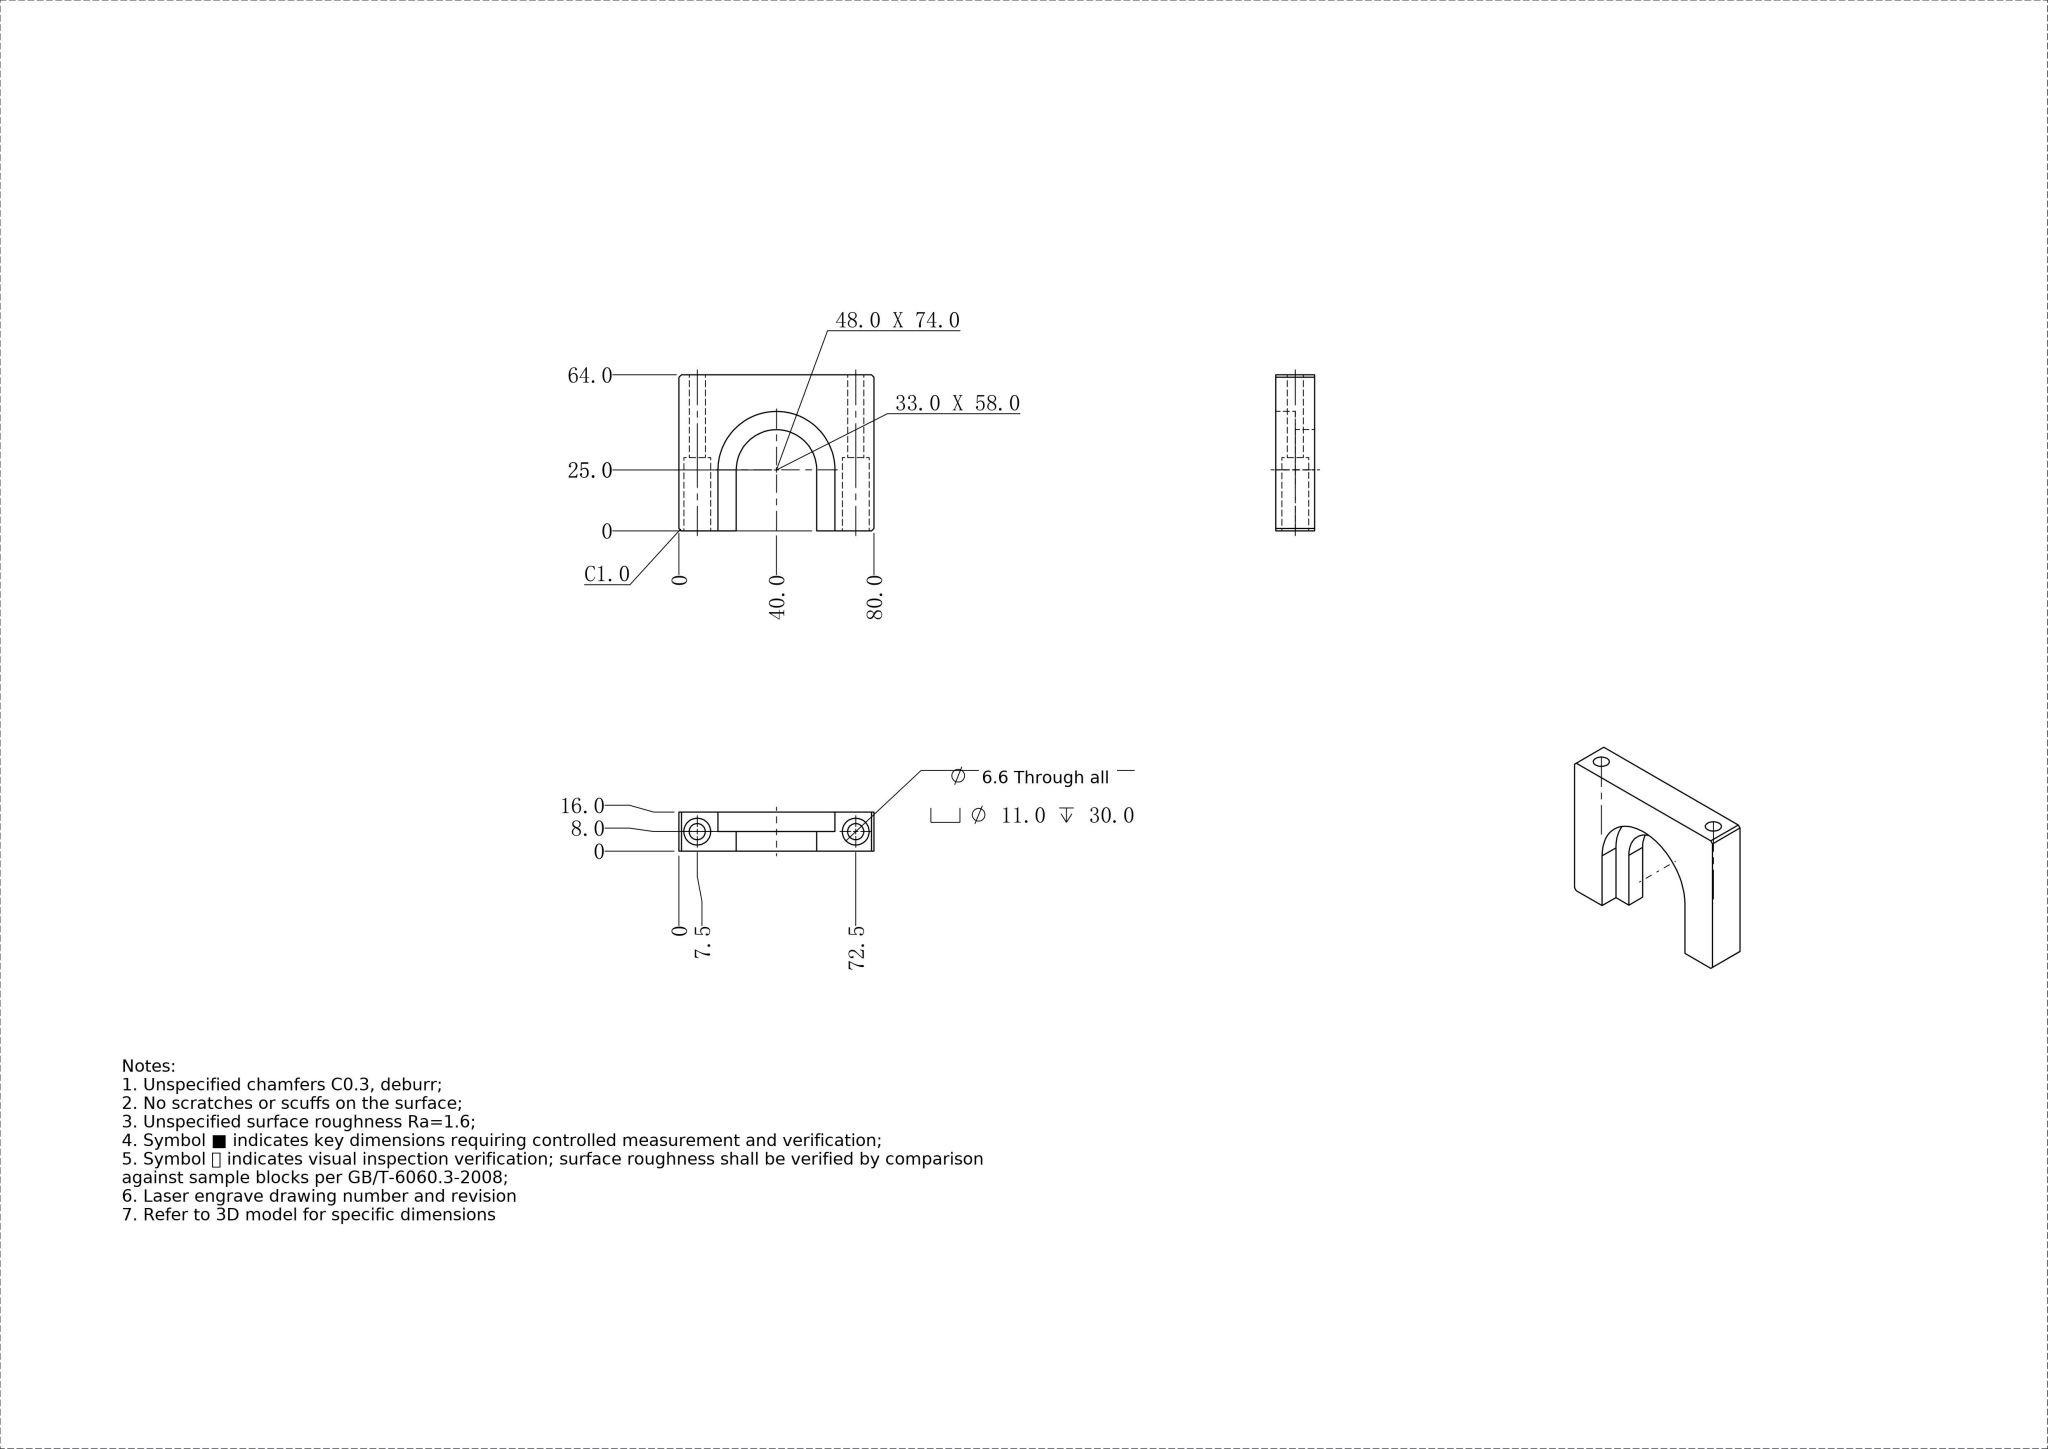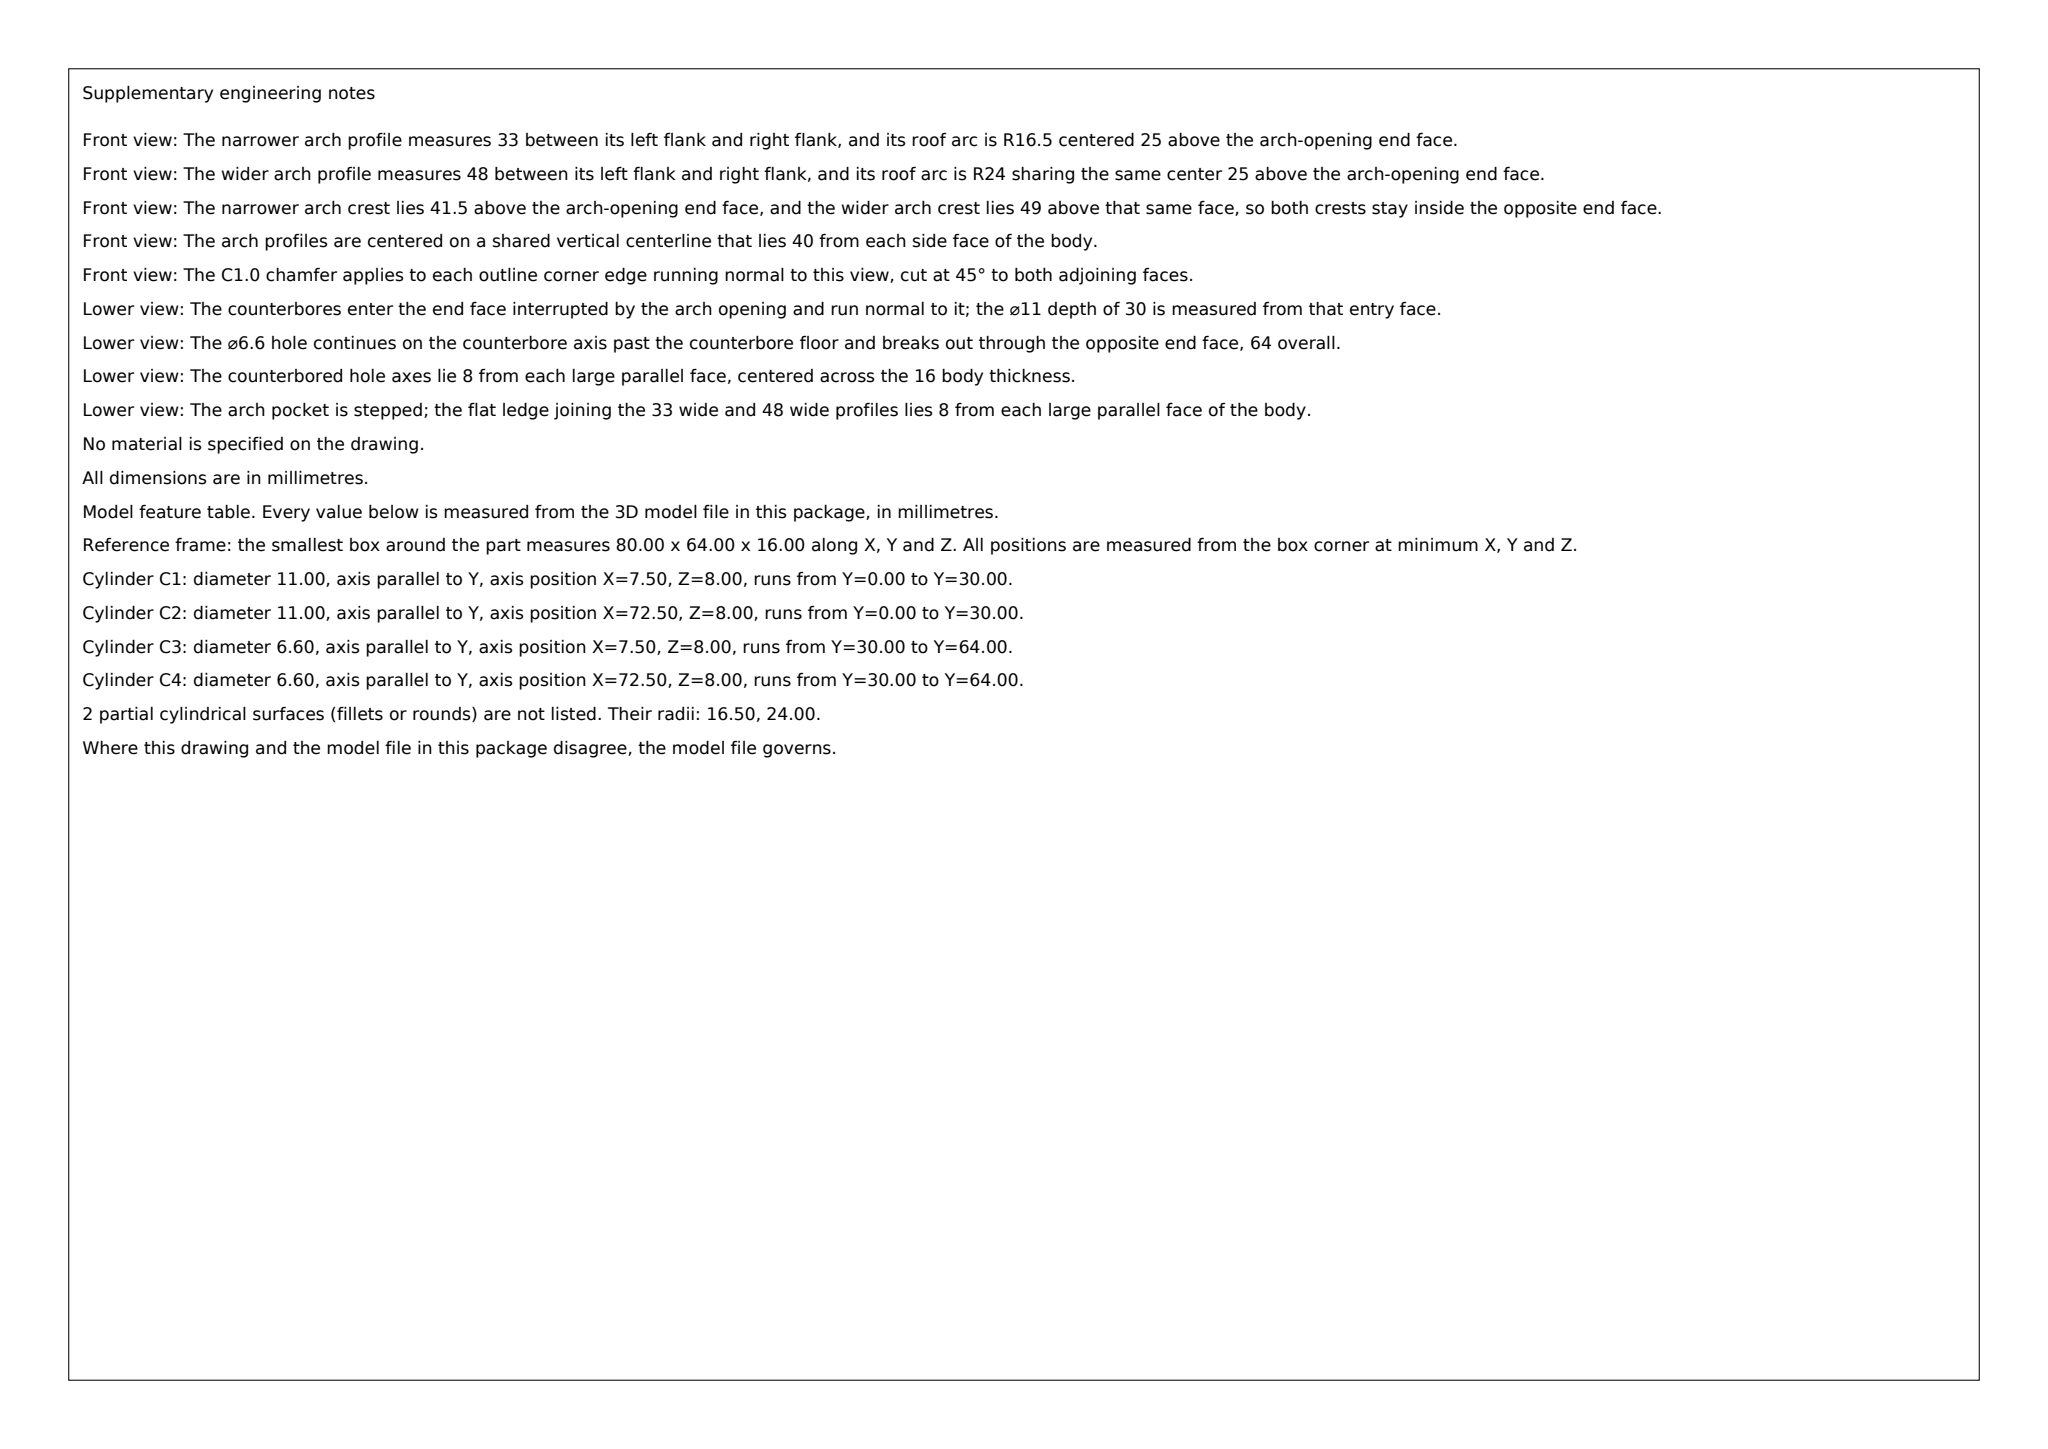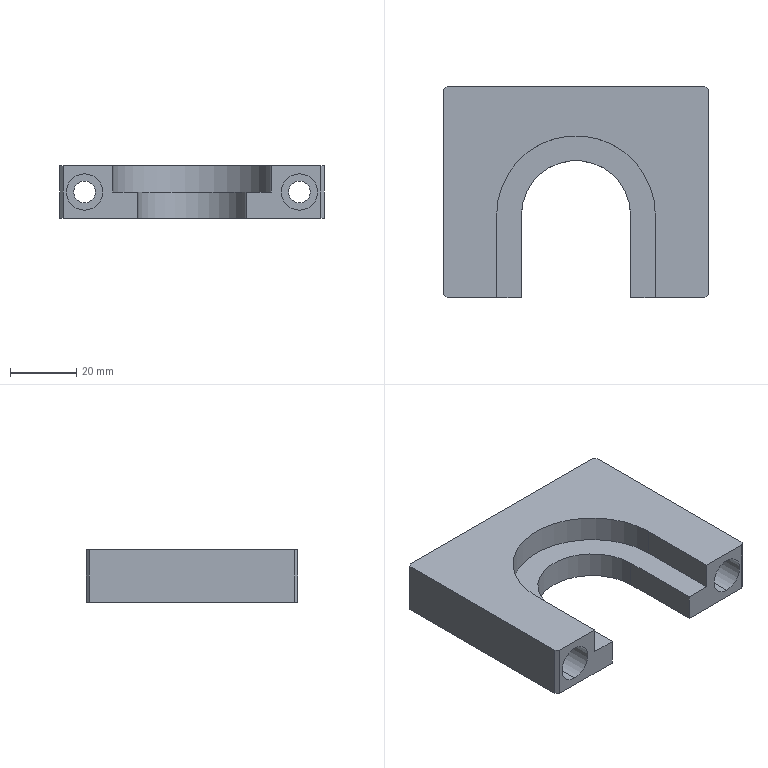Part | SolidWorks | mm | 1 solid | 28 faces | box 80 x 64 x 16 mm | volume 47000 mm3 | plane 18 | cylinder 10 | commonest cylinder face diameters 11 x4 6.6 x4 33 x1 48 x1
Drawing notes:
ALL DIMS IN MM UNLESS OTHERWISE NOTED | from the solid: STEP bbox 80.0 x 64.0 x 16.0 mm matches drawn 80.0/64.0/16.0 values
ARCH SLOTS Ø48.0 & Ø33.0 HT 8.0 EA, OPPOSITE FACES, THRU 16.0 | from the solid: cyl Ø48 axis z len 8 @ (40,25); cyl Ø33 axis z len 8 @ (40,25); z planes 0/8/16 in 16 thk plate
4X C1.0 CHAMFER ON ALL FOUR VERTICAL CORNER EDGES (AT X=0/80, Y=0/64), FULL 16.0 PART HEIGHT | from the solid: inclined_planes: four 45deg faces, size [1.0,1.0,16.0], bbox_from [0,0,0], [0,63,0], [79,0,0], [79,63,0]
build123d program:
from build123d import *

# Parameters (mm, degrees)
SKETCH1_W                                       = 80
SKETCH1_H                                       = 64
BOSS_EXTRUDE1_DEPTH                             = 16
CUT_EXTRUDE1_DEPTH                              = 16
CUT_EXTRUDE2_DEPTH                              = 8
M6_HEX_SOCKET_HEAD_CAP_SCREW_CBORE1_D           = 6.6
M6_HEX_SOCKET_HEAD_CAP_SCREW_CBORE1_CBORE_D     = 11
M6_HEX_SOCKET_HEAD_CAP_SCREW_CBORE1_CBORE_DEPTH = 30
CHAMFER1_SIZE                                   = 1


with BuildPart() as part:
    # Sketch1 → Boss-Extrude1 (new body)
    with BuildSketch(Plane.XY):
        Rectangle(SKETCH1_W, SKETCH1_H)
    extrude(amount=BOSS_EXTRUDE1_DEPTH)

    # Sketch2 → Cut-Extrude1 (cut)
    with BuildSketch(Plane.XY.offset(16)):
        with BuildLine():
            Line((-16.5, -32), (-16.5, -7))
            ThreePointArc((-16.5, -7), (0, 9.5), (16.5, -7))
            Line((16.5, -7), (16.5, -32))
            ThreePointArc((16.5, -32), (0, -48.5), (-16.5, -32))
        make_face()
    extrude(amount=-CUT_EXTRUDE1_DEPTH, mode=Mode.SUBTRACT)

    # Sketch3 → Cut-Extrude2 (cut)
    with BuildSketch(Plane.XY.offset(16)):
        with BuildLine():
            Line((24, -7), (24, -33))
            ThreePointArc((24, -33), (0, -57), (-24, -33))
            Line((-24, -33), (-24, -7))
            ThreePointArc((-24, -7), (0, 17), (24, -7))
        make_face()
    extrude(amount=-CUT_EXTRUDE2_DEPTH, mode=Mode.SUBTRACT)

    # M6 Hex Socket Head Cap Screw CBORE1 (through all)
    with Locations(Plane(origin=(0, -32, 0), x_dir=(-1, 0, 0), z_dir=(0, -1, 0))):
        with Locations((-32.5, -8), (32.5, -8)):
            CounterBoreHole(M6_HEX_SOCKET_HEAD_CAP_SCREW_CBORE1_D / 2, M6_HEX_SOCKET_HEAD_CAP_SCREW_CBORE1_CBORE_D / 2, M6_HEX_SOCKET_HEAD_CAP_SCREW_CBORE1_CBORE_DEPTH)

    # Chamfer1
    chamfer1_edges = [part.edges().sort_by_distance(p)[0] for p in [
        (40, -32, 8),
        (-40, -32, 8),
        (-40, 32, 8),
        (40, 32, 8),
    ]]
    chamfer(chamfer1_edges, length=CHAMFER1_SIZE)


solid = part.part
STEP:
#1=CARTESIAN_POINT('',(32.5,-2.,13.5));
#2=VERTEX_POINT('',#1);
#3=CARTESIAN_POINT('',(32.5,-2.,2.5));
#4=VERTEX_POINT('',#3);
#5=CARTESIAN_POINT('',(32.5,-2.,8.));
#6=DIRECTION('',(0.,-1.,0.));
#7=DIRECTION('',(0.,0.,-1.));
#8=AXIS2_PLACEMENT_3D('',#5,#6,#7);
#9=CIRCLE('',#8,5.5);
#10=EDGE_CURVE('',#2,#4,#9,.T.);
#11=ORIENTED_EDGE('',*,*,#10,.F.);
#12=CARTESIAN_POINT('',(32.5,-32.,13.5));
#13=VERTEX_POINT('',#12);
#14=CARTESIAN_POINT('',(32.5,-32.,13.5));
#15=DIRECTION('',(0.,-1.,0.));
#16=VECTOR('',#15,1000.);
#17=LINE('',#14,#16);
#18=EDGE_CURVE('',#2,#13,#17,.T.);
#19=ORIENTED_EDGE('',*,*,#18,.T.);
#20=CARTESIAN_POINT('',(32.5,-32.,2.5));
#21=VERTEX_POINT('',#20);
#22=CARTESIAN_POINT('',(32.5,-32.,8.));
#23=DIRECTION('',(0.,-1.,0.));
#24=DIRECTION('',(0.,0.,-1.));
#25=AXIS2_PLACEMENT_3D('',#22,#23,#24);
#26=CIRCLE('',#25,5.5);
#27=EDGE_CURVE('',#13,#21,#26,.T.);
#28=ORIENTED_EDGE('',*,*,#27,.T.);
#29=CARTESIAN_POINT('',(32.5,-32.,2.5));
#30=DIRECTION('',(0.,-1.,0.));
#31=VECTOR('',#30,1000.);
#32=LINE('',#29,#31);
#33=EDGE_CURVE('',#4,#21,#32,.T.);
#34=ORIENTED_EDGE('',*,*,#33,.F.);
#35=EDGE_LOOP('',(#11,#19,#28,#34));
#36=FACE_OUTER_BOUND('',#35,.T.);
#37=CARTESIAN_POINT('',(32.5,-32.,8.));
#38=DIRECTION('',(0.,-1.,0.));
#39=DIRECTION('',(0.,0.,-1.));
#40=AXIS2_PLACEMENT_3D('',#37,#38,#39);
#41=CYLINDRICAL_SURFACE('',#40,5.5);
#42=ADVANCED_FACE('',(#36),#41,.F.);
#43=CARTESIAN_POINT('',(32.5,32.,11.3));
#44=VERTEX_POINT('',#43);
#45=CARTESIAN_POINT('',(32.5,32.,4.7));
#46=VERTEX_POINT('',#45);
#47=CARTESIAN_POINT('',(32.5,32.,8.));
#48=DIRECTION('',(0.,-1.,0.));
#49=DIRECTION('',(0.,0.,-1.));
#50=AXIS2_PLACEMENT_3D('',#47,#48,#49);
#51=CIRCLE('',#50,3.3);
#52=EDGE_CURVE('',#44,#46,#51,.T.);
#53=ORIENTED_EDGE('',*,*,#52,.F.);
#54=CARTESIAN_POINT('',(32.5,-2.,11.3));
#55=VERTEX_POINT('',#54);
#56=CARTESIAN_POINT('',(32.5,-32.,11.3));
#57=DIRECTION('',(0.,-1.,0.));
#58=VECTOR('',#57,1000.);
#59=LINE('',#56,#58);
#60=EDGE_CURVE('',#44,#55,#59,.T.);
#61=ORIENTED_EDGE('',*,*,#60,.T.);
#62=CARTESIAN_POINT('',(32.5,-2.,4.7));
#63=VERTEX_POINT('',#62);
#64=CARTESIAN_POINT('',(32.5,-2.,8.));
#65=DIRECTION('',(0.,-1.,0.));
#66=DIRECTION('',(0.,0.,-1.));
#67=AXIS2_PLACEMENT_3D('',#64,#65,#66);
#68=CIRCLE('',#67,3.3);
#69=EDGE_CURVE('',#55,#63,#68,.T.);
#70=ORIENTED_EDGE('',*,*,#69,.T.);
#71=CARTESIAN_POINT('',(32.5,-32.,4.7));
#72=DIRECTION('',(0.,-1.,0.));
#73=VECTOR('',#72,1000.);
#74=LINE('',#71,#73);
#75=EDGE_CURVE('',#46,#63,#74,.T.);
#76=ORIENTED_EDGE('',*,*,#75,.F.);
#77=EDGE_LOOP('',(#53,#61,#70,#76));
#78=FACE_OUTER_BOUND('',#77,.T.);
#79=CARTESIAN_POINT('',(32.5,-32.,8.));
#80=DIRECTION('',(0.,-1.,0.));
#81=DIRECTION('',(0.,0.,-1.));
#82=AXIS2_PLACEMENT_3D('',#79,#80,#81);
#83=CYLINDRICAL_SURFACE('',#82,3.3);
#84=ADVANCED_FACE('',(#78),#83,.F.);
#85=CARTESIAN_POINT('',(-32.5,-2.,13.5));
#86=VERTEX_POINT('',#85);
#87=CARTESIAN_POINT('',(-32.5,-2.,2.5));
#88=VERTEX_POINT('',#87);
#89=CARTESIAN_POINT('',(-32.5,-2.,8.));
#90=DIRECTION('',(0.,-1.,0.));
#91=DIRECTION('',(0.,0.,-1.));
#92=AXIS2_PLACEMENT_3D('',#89,#90,#91);
#93=CIRCLE('',#92,5.5);
#94=EDGE_CURVE('',#86,#88,#93,.T.);
#95=ORIENTED_EDGE('',*,*,#94,.F.);
#96=CARTESIAN_POINT('',(-32.5,-32.,13.5));
#97=VERTEX_POINT('',#96);
#98=CARTESIAN_POINT('',(-32.5,-32.,13.5));
#99=DIRECTION('',(0.,-1.,0.));
#100=VECTOR('',#99,1000.);
#101=LINE('',#98,#100);
#102=EDGE_CURVE('',#86,#97,#101,.T.);
#103=ORIENTED_EDGE('',*,*,#102,.T.);
#104=CARTESIAN_POINT('',(-32.5,-32.,2.5));
#105=VERTEX_POINT('',#104);
#106=CARTESIAN_POINT('',(-32.5,-32.,8.));
#107=DIRECTION('',(0.,-1.,0.));
#108=DIRECTION('',(0.,0.,-1.));
#109=AXIS2_PLACEMENT_3D('',#106,#107,#108);
#110=CIRCLE('',#109,5.5);
#111=EDGE_CURVE('',#97,#105,#110,.T.);
#112=ORIENTED_EDGE('',*,*,#111,.T.);
#113=CARTESIAN_POINT('',(-32.5,-32.,2.5));
#114=DIRECTION('',(0.,-1.,0.));
#115=VECTOR('',#114,1000.);
#116=LINE('',#113,#115);
#117=EDGE_CURVE('',#88,#105,#116,.T.);
#118=ORIENTED_EDGE('',*,*,#117,.F.);
#119=EDGE_LOOP('',(#95,#103,#112,#118));
#120=FACE_OUTER_BOUND('',#119,.T.);
#121=CARTESIAN_POINT('',(-32.5,-32.,8.));
#122=DIRECTION('',(0.,-1.,0.));
#123=DIRECTION('',(0.,0.,-1.));
#124=AXIS2_PLACEMENT_3D('',#121,#122,#123);
#125=CYLINDRICAL_SURFACE('',#124,5.5);
#126=ADVANCED_FACE('',(#120),#125,.F.);
#127=CARTESIAN_POINT('',(-32.5,32.,11.3));
#128=VERTEX_POINT('',#127);
#129=CARTESIAN_POINT('',(-32.5,32.,4.7));
#130=VERTEX_POINT('',#129);
#131=CARTESIAN_POINT('',(-32.5,32.,8.));
#132=DIRECTION('',(0.,-1.,0.));
#133=DIRECTION('',(0.,0.,-1.));
#134=AXIS2_PLACEMENT_3D('',#131,#132,#133);
#135=CIRCLE('',#134,3.3);
#136=EDGE_CURVE('',#128,#130,#135,.T.);
#137=ORIENTED_EDGE('',*,*,#136,.F.);
#138=CARTESIAN_POINT('',(-32.5,-2.,11.3));
#139=VERTEX_POINT('',#138);
#140=CARTESIAN_POINT('',(-32.5,-32.,11.3));
#141=DIRECTION('',(0.,-1.,0.));
#142=VECTOR('',#141,1000.);
#143=LINE('',#140,#142);
#144=EDGE_CURVE('',#128,#139,#143,.T.);
#145=ORIENTED_EDGE('',*,*,#144,.T.);
#146=CARTESIAN_POINT('',(-32.5,-2.,4.7));
#147=VERTEX_POINT('',#146);
#148=CARTESIAN_POINT('',(-32.5,-2.,8.));
#149=DIRECTION('',(0.,-1.,0.));
#150=DIRECTION('',(0.,0.,-1.));
#151=AXIS2_PLACEMENT_3D('',#148,#149,#150);
#152=CIRCLE('',#151,3.3);
#153=EDGE_CURVE('',#139,#147,#152,.T.);
#154=ORIENTED_EDGE('',*,*,#153,.T.);
#155=CARTESIAN_POINT('',(-32.5,-32.,4.7));
#156=DIRECTION('',(0.,-1.,0.));
#157=VECTOR('',#156,1000.);
#158=LINE('',#155,#157);
#159=EDGE_CURVE('',#130,#147,#158,.T.);
#160=ORIENTED_EDGE('',*,*,#159,.F.);
#161=EDGE_LOOP('',(#137,#145,#154,#160));
#162=FACE_OUTER_BOUND('',#161,.T.);
#163=CARTESIAN_POINT('',(-32.5,-32.,8.));
#164=DIRECTION('',(0.,-1.,0.));
#165=DIRECTION('',(0.,0.,-1.));
#166=AXIS2_PLACEMENT_3D('',#163,#164,#165);
#167=CYLINDRICAL_SURFACE('',#166,3.3);
#168=ADVANCED_FACE('',(#162),#167,.F.);
#169=CARTESIAN_POINT('',(-16.5,-32.,8.));
#170=VERTEX_POINT('',#169);
#171=CARTESIAN_POINT('',(-16.5,-7.,8.));
#172=VERTEX_POINT('',#171);
#173=CARTESIAN_POINT('',(-16.5,-32.,8.));
#174=DIRECTION('',(0.,1.,0.));
#175=VECTOR('',#174,1000.);
#176=LINE('',#173,#175);
#177=EDGE_CURVE('',#170,#172,#176,.T.);
#178=ORIENTED_EDGE('',*,*,#177,.F.);
#179=CARTESIAN_POINT('',(-16.5,-32.,0.));
#180=VERTEX_POINT('',#179);
#181=CARTESIAN_POINT('',(-16.5,-32.,0.));
#182=DIRECTION('',(0.,0.,1.));
#183=VECTOR('',#182,1000.);
#184=LINE('',#181,#183);
#185=EDGE_CURVE('',#180,#170,#184,.T.);
#186=ORIENTED_EDGE('',*,*,#185,.F.);
#187=CARTESIAN_POINT('',(-16.5,-7.,0.));
#188=VERTEX_POINT('',#187);
#189=CARTESIAN_POINT('',(-16.5,-32.,0.));
#190=DIRECTION('',(0.,-1.,0.));
#191=VECTOR('',#190,1000.);
#192=LINE('',#189,#191);
#193=EDGE_CURVE('',#188,#180,#192,.T.);
#194=ORIENTED_EDGE('',*,*,#193,.F.);
#195=CARTESIAN_POINT('',(-16.5,-7.,0.));
#196=DIRECTION('',(0.,0.,1.));
#197=VECTOR('',#196,1000.);
#198=LINE('',#195,#197);
#199=EDGE_CURVE('',#188,#172,#198,.T.);
#200=ORIENTED_EDGE('',*,*,#199,.T.);
#201=EDGE_LOOP('',(#178,#186,#194,#200));
#202=FACE_OUTER_BOUND('',#201,.T.);
#203=CARTESIAN_POINT('',(-16.5,-32.,0.));
#204=DIRECTION('',(-1.,0.,0.));
#205=DIRECTION('',(0.,0.,1.));
#206=AXIS2_PLACEMENT_3D('',#203,#204,#205);
#207=PLANE('',#206);
#208=ADVANCED_FACE('',(#202),#207,.F.);
#209=CARTESIAN_POINT('',(16.5,-7.,8.));
#210=VERTEX_POINT('',#209);
#211=CARTESIAN_POINT('',(0.,-7.,8.));
#212=DIRECTION('',(0.,0.,-1.));
#213=DIRECTION('',(1.,0.,0.));
#214=AXIS2_PLACEMENT_3D('',#211,#212,#213);
#215=CIRCLE('',#214,16.5);
#216=EDGE_CURVE('',#172,#210,#215,.T.);
#217=ORIENTED_EDGE('',*,*,#216,.F.);
#218=ORIENTED_EDGE('',*,*,#199,.F.);
#219=CARTESIAN_POINT('',(16.5,-7.,0.));
#220=VERTEX_POINT('',#219);
#221=CARTESIAN_POINT('',(0.,-7.,0.));
#222=DIRECTION('',(0.,0.,1.));
#223=DIRECTION('',(1.,0.,0.));
#224=AXIS2_PLACEMENT_3D('',#221,#222,#223);
#225=CIRCLE('',#224,16.5);
#226=EDGE_CURVE('',#220,#188,#225,.T.);
#227=ORIENTED_EDGE('',*,*,#226,.F.);
#228=CARTESIAN_POINT('',(16.5,-7.,0.));
#229=DIRECTION('',(0.,0.,1.));
#230=VECTOR('',#229,1000.);
#231=LINE('',#228,#230);
#232=EDGE_CURVE('',#220,#210,#231,.T.);
#233=ORIENTED_EDGE('',*,*,#232,.T.);
#234=EDGE_LOOP('',(#217,#218,#227,#233));
#235=FACE_OUTER_BOUND('',#234,.T.);
#236=CARTESIAN_POINT('',(0.,-7.,0.));
#237=DIRECTION('',(0.,0.,1.));
#238=DIRECTION('',(1.,0.,0.));
#239=AXIS2_PLACEMENT_3D('',#236,#237,#238);
#240=CYLINDRICAL_SURFACE('',#239,16.5);
#241=ADVANCED_FACE('',(#235),#240,.F.);
#242=CARTESIAN_POINT('',(16.5,-32.,8.));
#243=VERTEX_POINT('',#242);
#244=CARTESIAN_POINT('',(16.5,-32.,8.));
#245=DIRECTION('',(0.,-1.,0.));
#246=VECTOR('',#245,1000.);
#247=LINE('',#244,#246);
#248=EDGE_CURVE('',#210,#243,#247,.T.);
#249=ORIENTED_EDGE('',*,*,#248,.F.);
#250=ORIENTED_EDGE('',*,*,#232,.F.);
#251=CARTESIAN_POINT('',(16.5,-32.,0.));
#252=VERTEX_POINT('',#251);
#253=CARTESIAN_POINT('',(16.5,-32.,0.));
#254=DIRECTION('',(0.,1.,0.));
#255=VECTOR('',#254,1000.);
#256=LINE('',#253,#255);
#257=EDGE_CURVE('',#252,#220,#256,.T.);
#258=ORIENTED_EDGE('',*,*,#257,.F.);
#259=CARTESIAN_POINT('',(16.5,-32.,0.));
#260=DIRECTION('',(0.,0.,1.));
#261=VECTOR('',#260,1000.);
#262=LINE('',#259,#261);
#263=EDGE_CURVE('',#252,#243,#262,.T.);
#264=ORIENTED_EDGE('',*,*,#263,.T.);
#265=EDGE_LOOP('',(#249,#250,#258,#264));
#266=FACE_OUTER_BOUND('',#265,.T.);
#267=CARTESIAN_POINT('',(16.5,-32.,0.));
#268=DIRECTION('',(1.,0.,0.));
#269=DIRECTION('',(0.,0.,-1.));
#270=AXIS2_PLACEMENT_3D('',#267,#268,#269);
#271=PLANE('',#270);
#272=ADVANCED_FACE('',(#266),#271,.F.);
#273=CARTESIAN_POINT('',(-32.5,-32.,8.));
#274=DIRECTION('',(0.,-1.,0.));
#275=DIRECTION('',(0.,0.,-1.));
#276=AXIS2_PLACEMENT_3D('',#273,#274,#275);
#277=CIRCLE('',#276,5.5);
#278=EDGE_CURVE('',#105,#97,#277,.T.);
#279=ORIENTED_EDGE('',*,*,#278,.F.);
#280=ORIENTED_EDGE('',*,*,#111,.F.);
#281=EDGE_LOOP('',(#279,#280));
#282=FACE_BOUND('',#281,.T.);
#283=CARTESIAN_POINT('',(-39.,-32.,16.));
#284=VERTEX_POINT('',#283);
#285=CARTESIAN_POINT('',(-24.,-32.,16.));
#286=VERTEX_POINT('',#285);
#287=CARTESIAN_POINT('',(-40.,-32.,16.));
#288=DIRECTION('',(1.,0.,0.));
#289=VECTOR('',#288,1000.);
#290=LINE('',#287,#289);
#291=EDGE_CURVE('',#284,#286,#290,.T.);
#292=ORIENTED_EDGE('',*,*,#291,.F.);
#293=CARTESIAN_POINT('',(-39.,-32.,0.));
#294=VERTEX_POINT('',#293);
#295=CARTESIAN_POINT('',(-39.,-32.,16.));
#296=DIRECTION('',(0.,0.,-1.));
#297=VECTOR('',#296,1000.);
#298=LINE('',#295,#297);
#299=EDGE_CURVE('',#284,#294,#298,.T.);
#300=ORIENTED_EDGE('',*,*,#299,.T.);
#301=CARTESIAN_POINT('',(-40.,-32.,0.));
#302=DIRECTION('',(1.,0.,0.));
#303=VECTOR('',#302,1000.);
#304=LINE('',#301,#303);
#305=EDGE_CURVE('',#294,#180,#304,.T.);
#306=ORIENTED_EDGE('',*,*,#305,.T.);
#307=ORIENTED_EDGE('',*,*,#185,.T.);
#308=CARTESIAN_POINT('',(-24.,-32.,8.));
#309=VERTEX_POINT('',#308);
#310=CARTESIAN_POINT('',(-40.,-32.,8.));
#311=DIRECTION('',(1.,0.,0.));
#312=VECTOR('',#311,1000.);
#313=LINE('',#310,#312);
#314=EDGE_CURVE('',#309,#170,#313,.T.);
#315=ORIENTED_EDGE('',*,*,#314,.F.);
#316=CARTESIAN_POINT('',(-24.,-32.,16.));
#317=DIRECTION('',(0.,0.,1.));
#318=VECTOR('',#317,1000.);
#319=LINE('',#316,#318);
#320=EDGE_CURVE('',#309,#286,#319,.T.);
#321=ORIENTED_EDGE('',*,*,#320,.T.);
#322=EDGE_LOOP('',(#292,#300,#306,#307,#315,#321));
#323=FACE_OUTER_BOUND('',#322,.T.);
#324=CARTESIAN_POINT('',(-40.,-32.,16.));
#325=DIRECTION('',(0.,1.,0.));
#326=DIRECTION('',(0.,0.,1.));
#327=AXIS2_PLACEMENT_3D('',#324,#325,#326);
#328=PLANE('',#327);
#329=ADVANCED_FACE('',(#282,#323),#328,.F.);
#330=CARTESIAN_POINT('',(40.,-31.,16.));
#331=VERTEX_POINT('',#330);
#332=CARTESIAN_POINT('',(40.,31.,16.));
#333=VERTEX_POINT('',#332);
#334=CARTESIAN_POINT('',(40.,32.,16.));
#335=DIRECTION('',(0.,1.,0.));
#336=VECTOR('',#335,1000.);
#337=LINE('',#334,#336);
#338=EDGE_CURVE('',#331,#333,#337,.T.);
#339=ORIENTED_EDGE('',*,*,#338,.F.);
#340=CARTESIAN_POINT('',(40.,-31.,0.));
#341=VERTEX_POINT('',#340);
#342=CARTESIAN_POINT('',(40.,-31.,16.));
#343=DIRECTION('',(0.,0.,-1.));
#344=VECTOR('',#343,1000.);
#345=LINE('',#342,#344);
#346=EDGE_CURVE('',#331,#341,#345,.T.);
#347=ORIENTED_EDGE('',*,*,#346,.T.);
#348=CARTESIAN_POINT('',(40.,31.,0.));
#349=VERTEX_POINT('',#348);
#350=CARTESIAN_POINT('',(40.,32.,0.));
#351=DIRECTION('',(0.,1.,0.));
#352=VECTOR('',#351,1000.);
#353=LINE('',#350,#352);
#354=EDGE_CURVE('',#341,#349,#353,.T.);
#355=ORIENTED_EDGE('',*,*,#354,.T.);
#356=CARTESIAN_POINT('',(40.,31.,16.));
#357=DIRECTION('',(0.,0.,1.));
#358=VECTOR('',#357,1000.);
#359=LINE('',#356,#358);
#360=EDGE_CURVE('',#349,#333,#359,.T.);
#361=ORIENTED_EDGE('',*,*,#360,.T.);
#362=EDGE_LOOP('',(#339,#347,#355,#361));
#363=FACE_OUTER_BOUND('',#362,.T.);
#364=CARTESIAN_POINT('',(40.,32.,16.));
#365=DIRECTION('',(-1.,0.,0.));
#366=DIRECTION('',(0.,0.,1.));
#367=AXIS2_PLACEMENT_3D('',#364,#365,#366);
#368=PLANE('',#367);
#369=ADVANCED_FACE('',(#363),#368,.F.);
#370=CARTESIAN_POINT('',(32.5,32.,8.));
#371=DIRECTION('',(0.,-1.,0.));
#372=DIRECTION('',(0.,0.,-1.));
#373=AXIS2_PLACEMENT_3D('',#370,#371,#372);
#374=CIRCLE('',#373,3.3);
#375=EDGE_CURVE('',#46,#44,#374,.T.);
#376=ORIENTED_EDGE('',*,*,#375,.T.);
#377=ORIENTED_EDGE('',*,*,#52,.T.);
#378=EDGE_LOOP('',(#376,#377));
#379=FACE_BOUND('',#378,.T.);
#380=CARTESIAN_POINT('',(-32.5,32.,8.));
#381=DIRECTION('',(0.,-1.,0.));
#382=DIRECTION('',(0.,0.,-1.));
#383=AXIS2_PLACEMENT_3D('',#380,#381,#382);
#384=CIRCLE('',#383,3.3);
#385=EDGE_CURVE('',#130,#128,#384,.T.);
#386=ORIENTED_EDGE('',*,*,#385,.T.);
#387=ORIENTED_EDGE('',*,*,#136,.T.);
#388=EDGE_LOOP('',(#386,#387));
#389=FACE_BOUND('',#388,.T.);
#390=CARTESIAN_POINT('',(39.,32.,0.));
#391=VERTEX_POINT('',#390);
#392=CARTESIAN_POINT('',(-39.,32.,0.));
#393=VERTEX_POINT('',#392);
#394=CARTESIAN_POINT('',(-40.,32.,0.));
#395=DIRECTION('',(-1.,0.,0.));
#396=VECTOR('',#395,1000.);
#397=LINE('',#394,#396);
#398=EDGE_CURVE('',#391,#393,#397,.T.);
#399=ORIENTED_EDGE('',*,*,#398,.T.);
#400=CARTESIAN_POINT('',(-39.,32.,16.));
#401=VERTEX_POINT('',#400);
#402=CARTESIAN_POINT('',(-39.,32.,16.));
#403=DIRECTION('',(0.,0.,1.));
#404=VECTOR('',#403,1000.);
#405=LINE('',#402,#404);
#406=EDGE_CURVE('',#393,#401,#405,.T.);
#407=ORIENTED_EDGE('',*,*,#406,.T.);
#408=CARTESIAN_POINT('',(39.,32.,16.));
#409=VERTEX_POINT('',#408);
#410=CARTESIAN_POINT('',(-40.,32.,16.));
#411=DIRECTION('',(-1.,0.,0.));
#412=VECTOR('',#411,1000.);
#413=LINE('',#410,#412);
#414=EDGE_CURVE('',#409,#401,#413,.T.);
#415=ORIENTED_EDGE('',*,*,#414,.F.);
#416=CARTESIAN_POINT('',(39.,32.,16.));
#417=DIRECTION('',(0.,0.,-1.));
#418=VECTOR('',#417,1000.);
#419=LINE('',#416,#418);
#420=EDGE_CURVE('',#409,#391,#419,.T.);
#421=ORIENTED_EDGE('',*,*,#420,.T.);
#422=EDGE_LOOP('',(#399,#407,#415,#421));
#423=FACE_OUTER_BOUND('',#422,.T.);
#424=CARTESIAN_POINT('',(-40.,32.,16.));
#425=DIRECTION('',(0.,-1.,0.));
#426=DIRECTION('',(0.,0.,-1.));
#427=AXIS2_PLACEMENT_3D('',#424,#425,#426);
#428=PLANE('',#427);
#429=ADVANCED_FACE('',(#379,#389,#423),#428,.F.);
#430=CARTESIAN_POINT('',(-40.,31.,0.));
#431=VERTEX_POINT('',#430);
#432=CARTESIAN_POINT('',(-40.,-31.,0.));
#433=VERTEX_POINT('',#432);
#434=CARTESIAN_POINT('',(-40.,32.,0.));
#435=DIRECTION('',(-0.,-1.,0.));
#436=VECTOR('',#435,1000.);
#437=LINE('',#434,#436);
#438=EDGE_CURVE('',#431,#433,#437,.T.);
#439=ORIENTED_EDGE('',*,*,#438,.T.);
#440=CARTESIAN_POINT('',(-40.,-31.,16.));
#441=VERTEX_POINT('',#440);
#442=CARTESIAN_POINT('',(-40.,-31.,16.));
#443=DIRECTION('',(0.,0.,1.));
#444=VECTOR('',#443,1000.);
#445=LINE('',#442,#444);
#446=EDGE_CURVE('',#433,#441,#445,.T.);
#447=ORIENTED_EDGE('',*,*,#446,.T.);
#448=CARTESIAN_POINT('',(-40.,31.,16.));
#449=VERTEX_POINT('',#448);
#450=CARTESIAN_POINT('',(-40.,32.,16.));
#451=DIRECTION('',(-0.,-1.,0.));
#452=VECTOR('',#451,1000.);
#453=LINE('',#450,#452);
#454=EDGE_CURVE('',#449,#441,#453,.T.);
#455=ORIENTED_EDGE('',*,*,#454,.F.);
#456=CARTESIAN_POINT('',(-40.,31.,16.));
#457=DIRECTION('',(0.,0.,-1.));
#458=VECTOR('',#457,1000.);
#459=LINE('',#456,#458);
#460=EDGE_CURVE('',#449,#431,#459,.T.);
#461=ORIENTED_EDGE('',*,*,#460,.T.);
#462=EDGE_LOOP('',(#439,#447,#455,#461));
#463=FACE_OUTER_BOUND('',#462,.T.);
#464=CARTESIAN_POINT('',(-40.,32.,16.));
#465=DIRECTION('',(1.,-0.,0.));
#466=DIRECTION('',(0.,1.,0.));
#467=AXIS2_PLACEMENT_3D('',#464,#465,#466);
#468=PLANE('',#467);
#469=ADVANCED_FACE('',(#463),#468,.F.);
#470=CARTESIAN_POINT('',(32.5,-32.,8.));
#471=DIRECTION('',(0.,-1.,0.));
#472=DIRECTION('',(0.,0.,-1.));
#473=AXIS2_PLACEMENT_3D('',#470,#471,#472);
#474=CIRCLE('',#473,5.5);
#475=EDGE_CURVE('',#21,#13,#474,.T.);
#476=ORIENTED_EDGE('',*,*,#475,.F.);
#477=ORIENTED_EDGE('',*,*,#27,.F.);
#478=EDGE_LOOP('',(#476,#477));
#479=FACE_BOUND('',#478,.T.);
#480=CARTESIAN_POINT('',(39.,-32.,0.));
#481=VERTEX_POINT('',#480);
#482=CARTESIAN_POINT('',(-40.,-32.,0.));
#483=DIRECTION('',(1.,0.,0.));
#484=VECTOR('',#483,1000.);
#485=LINE('',#482,#484);
#486=EDGE_CURVE('',#252,#481,#485,.T.);
#487=ORIENTED_EDGE('',*,*,#486,.T.);
#488=CARTESIAN_POINT('',(39.,-32.,16.));
#489=VERTEX_POINT('',#488);
#490=CARTESIAN_POINT('',(39.,-32.,16.));
#491=DIRECTION('',(0.,0.,1.));
#492=VECTOR('',#491,1000.);
#493=LINE('',#490,#492);
#494=EDGE_CURVE('',#481,#489,#493,.T.);
#495=ORIENTED_EDGE('',*,*,#494,.T.);
#496=CARTESIAN_POINT('',(24.,-32.,16.));
#497=VERTEX_POINT('',#496);
#498=CARTESIAN_POINT('',(-40.,-32.,16.));
#499=DIRECTION('',(1.,0.,0.));
#500=VECTOR('',#499,1000.);
#501=LINE('',#498,#500);
#502=EDGE_CURVE('',#497,#489,#501,.T.);
#503=ORIENTED_EDGE('',*,*,#502,.F.);
#504=CARTESIAN_POINT('',(24.,-32.,8.));
#505=VERTEX_POINT('',#504);
#506=CARTESIAN_POINT('',(24.,-32.,16.));
#507=DIRECTION('',(0.,0.,-1.));
#508=VECTOR('',#507,1000.);
#509=LINE('',#506,#508);
#510=EDGE_CURVE('',#497,#505,#509,.T.);
#511=ORIENTED_EDGE('',*,*,#510,.T.);
#512=CARTESIAN_POINT('',(-40.,-32.,8.));
#513=DIRECTION('',(1.,0.,0.));
#514=VECTOR('',#513,1000.);
#515=LINE('',#512,#514);
#516=EDGE_CURVE('',#243,#505,#515,.T.);
#517=ORIENTED_EDGE('',*,*,#516,.F.);
#518=ORIENTED_EDGE('',*,*,#263,.F.);
#519=EDGE_LOOP('',(#487,#495,#503,#511,#517,#518));
#520=FACE_OUTER_BOUND('',#519,.T.);
#521=CARTESIAN_POINT('',(-40.,-32.,16.));
#522=DIRECTION('',(0.,1.,0.));
#523=DIRECTION('',(0.,0.,1.));
#524=AXIS2_PLACEMENT_3D('',#521,#522,#523);
#525=PLANE('',#524);
#526=ADVANCED_FACE('',(#479,#520),#525,.F.);
#527=ORIENTED_EDGE('',*,*,#502,.T.);
#528=CARTESIAN_POINT('',(35.5,-35.5,16.));
#529=DIRECTION('',(0.7071,0.7071,0.));
#530=VECTOR('',#529,1000.);
#531=LINE('',#528,#530);
#532=EDGE_CURVE('',#489,#331,#531,.T.);
#533=ORIENTED_EDGE('',*,*,#532,.T.);
#534=ORIENTED_EDGE('',*,*,#338,.T.);
#535=CARTESIAN_POINT('',(35.5,35.5,16.));
#536=DIRECTION('',(-0.7071,0.7071,0.));
#537=VECTOR('',#536,1000.);
#538=LINE('',#535,#537);
#539=EDGE_CURVE('',#333,#409,#538,.T.);
#540=ORIENTED_EDGE('',*,*,#539,.T.);
#541=ORIENTED_EDGE('',*,*,#414,.T.);
#542=CARTESIAN_POINT('',(-35.5,35.5,16.));
#543=DIRECTION('',(-0.7071,-0.7071,0.));
#544=VECTOR('',#543,1000.);
#545=LINE('',#542,#544);
#546=EDGE_CURVE('',#401,#449,#545,.T.);
#547=ORIENTED_EDGE('',*,*,#546,.T.);
#548=ORIENTED_EDGE('',*,*,#454,.T.);
#549=CARTESIAN_POINT('',(-35.5,-35.5,16.));
#550=DIRECTION('',(0.7071,-0.7071,0.));
#551=VECTOR('',#550,1000.);
#552=LINE('',#549,#551);
#553=EDGE_CURVE('',#441,#284,#552,.T.);
#554=ORIENTED_EDGE('',*,*,#553,.T.);
#555=ORIENTED_EDGE('',*,*,#291,.T.);
#556=CARTESIAN_POINT('',(-24.,-7.,16.));
#557=VERTEX_POINT('',#556);
#558=CARTESIAN_POINT('',(-24.,-7.,16.));
#559=DIRECTION('',(0.,-1.,0.));
#560=VECTOR('',#559,1000.);
#561=LINE('',#558,#560);
#562=EDGE_CURVE('',#557,#286,#561,.T.);
#563=ORIENTED_EDGE('',*,*,#562,.F.);
#564=CARTESIAN_POINT('',(24.,-7.,16.));
#565=VERTEX_POINT('',#564);
#566=CARTESIAN_POINT('',(0.,-7.,16.));
#567=DIRECTION('',(0.,0.,1.));
#568=DIRECTION('',(1.,0.,0.));
#569=AXIS2_PLACEMENT_3D('',#566,#567,#568);
#570=CIRCLE('',#569,24.);
#571=EDGE_CURVE('',#565,#557,#570,.T.);
#572=ORIENTED_EDGE('',*,*,#571,.F.);
#573=CARTESIAN_POINT('',(24.,-7.,16.));
#574=DIRECTION('',(-0.,1.,0.));
#575=VECTOR('',#574,1000.);
#576=LINE('',#573,#575);
#577=EDGE_CURVE('',#497,#565,#576,.T.);
#578=ORIENTED_EDGE('',*,*,#577,.F.);
#579=EDGE_LOOP('',(#527,#533,#534,#540,#541,#547,#548,#554,#555,#563,#572,#578));
#580=FACE_OUTER_BOUND('',#579,.T.);
#581=CARTESIAN_POINT('',(0.,0.,16.));
#582=DIRECTION('',(0.,0.,1.));
#583=DIRECTION('',(1.,0.,0.));
#584=AXIS2_PLACEMENT_3D('',#581,#582,#583);
#585=PLANE('',#584);
#586=ADVANCED_FACE('',(#580),#585,.T.);
#587=ORIENTED_EDGE('',*,*,#354,.F.);
#588=CARTESIAN_POINT('',(40.,-31.,0.));
#589=DIRECTION('',(-0.7071,-0.7071,0.));
#590=VECTOR('',#589,1000.);
#591=LINE('',#588,#590);
#592=EDGE_CURVE('',#341,#481,#591,.T.);
#593=ORIENTED_EDGE('',*,*,#592,.T.);
#594=ORIENTED_EDGE('',*,*,#486,.F.);
#595=ORIENTED_EDGE('',*,*,#257,.T.);
#596=ORIENTED_EDGE('',*,*,#226,.T.);
#597=ORIENTED_EDGE('',*,*,#193,.T.);
#598=ORIENTED_EDGE('',*,*,#305,.F.);
#599=CARTESIAN_POINT('',(-39.,-32.,0.));
#600=DIRECTION('',(-0.7071,0.7071,0.));
#601=VECTOR('',#600,1000.);
#602=LINE('',#599,#601);
#603=EDGE_CURVE('',#294,#433,#602,.T.);
#604=ORIENTED_EDGE('',*,*,#603,.T.);
#605=ORIENTED_EDGE('',*,*,#438,.F.);
#606=CARTESIAN_POINT('',(-40.,31.,0.));
#607=DIRECTION('',(0.7071,0.7071,0.));
#608=VECTOR('',#607,1000.);
#609=LINE('',#606,#608);
#610=EDGE_CURVE('',#431,#393,#609,.T.);
#611=ORIENTED_EDGE('',*,*,#610,.T.);
#612=ORIENTED_EDGE('',*,*,#398,.F.);
#613=CARTESIAN_POINT('',(39.,32.,0.));
#614=DIRECTION('',(0.7071,-0.7071,0.));
#615=VECTOR('',#614,1000.);
#616=LINE('',#613,#615);
#617=EDGE_CURVE('',#391,#349,#616,.T.);
#618=ORIENTED_EDGE('',*,*,#617,.T.);
#619=EDGE_LOOP('',(#587,#593,#594,#595,#596,#597,#598,#604,#605,#611,#612,#618));
#620=FACE_OUTER_BOUND('',#619,.T.);
#621=CARTESIAN_POINT('',(0.,0.,0.));
#622=DIRECTION('',(0.,0.,1.));
#623=DIRECTION('',(1.,0.,0.));
#624=AXIS2_PLACEMENT_3D('',#621,#622,#623);
#625=PLANE('',#624);
#626=ADVANCED_FACE('',(#620),#625,.F.);
#627=ORIENTED_EDGE('',*,*,#577,.T.);
#628=CARTESIAN_POINT('',(24.,-7.,8.));
#629=VERTEX_POINT('',#628);
#630=CARTESIAN_POINT('',(24.,-7.,8.));
#631=DIRECTION('',(0.,0.,1.));
#632=VECTOR('',#631,1000.);
#633=LINE('',#630,#632);
#634=EDGE_CURVE('',#629,#565,#633,.T.);
#635=ORIENTED_EDGE('',*,*,#634,.F.);
#636=CARTESIAN_POINT('',(24.,-7.,8.));
#637=DIRECTION('',(-0.,1.,0.));
#638=VECTOR('',#637,1000.);
#639=LINE('',#636,#638);
#640=EDGE_CURVE('',#505,#629,#639,.T.);
#641=ORIENTED_EDGE('',*,*,#640,.F.);
#642=ORIENTED_EDGE('',*,*,#510,.F.);
#643=EDGE_LOOP('',(#627,#635,#641,#642));
#644=FACE_OUTER_BOUND('',#643,.T.);
#645=CARTESIAN_POINT('',(24.,-7.,8.));
#646=DIRECTION('',(1.,0.,0.));
#647=DIRECTION('',(-0.,1.,0.));
#648=AXIS2_PLACEMENT_3D('',#645,#646,#647);
#649=PLANE('',#648);
#650=ADVANCED_FACE('',(#644),#649,.F.);
#651=CARTESIAN_POINT('',(-24.,-7.,8.));
#652=VERTEX_POINT('',#651);
#653=CARTESIAN_POINT('',(-24.,-7.,8.));
#654=DIRECTION('',(0.,-1.,0.));
#655=VECTOR('',#654,1000.);
#656=LINE('',#653,#655);
#657=EDGE_CURVE('',#652,#309,#656,.T.);
#658=ORIENTED_EDGE('',*,*,#657,.F.);
#659=CARTESIAN_POINT('',(-24.,-7.,8.));
#660=DIRECTION('',(0.,0.,1.));
#661=VECTOR('',#660,1000.);
#662=LINE('',#659,#661);
#663=EDGE_CURVE('',#652,#557,#662,.T.);
#664=ORIENTED_EDGE('',*,*,#663,.T.);
#665=ORIENTED_EDGE('',*,*,#562,.T.);
#666=ORIENTED_EDGE('',*,*,#320,.F.);
#667=EDGE_LOOP('',(#658,#664,#665,#666));
#668=FACE_OUTER_BOUND('',#667,.T.);
#669=CARTESIAN_POINT('',(-24.,-7.,8.));
#670=DIRECTION('',(-1.,0.,0.));
#671=DIRECTION('',(0.,0.,1.));
#672=AXIS2_PLACEMENT_3D('',#669,#670,#671);
#673=PLANE('',#672);
#674=ADVANCED_FACE('',(#668),#673,.F.);
#675=ORIENTED_EDGE('',*,*,#314,.T.);
#676=ORIENTED_EDGE('',*,*,#177,.T.);
#677=ORIENTED_EDGE('',*,*,#216,.T.);
#678=ORIENTED_EDGE('',*,*,#248,.T.);
#679=ORIENTED_EDGE('',*,*,#516,.T.);
#680=ORIENTED_EDGE('',*,*,#640,.T.);
#681=CARTESIAN_POINT('',(0.,-7.,8.));
#682=DIRECTION('',(0.,0.,1.));
#683=DIRECTION('',(1.,0.,0.));
#684=AXIS2_PLACEMENT_3D('',#681,#682,#683);
#685=CIRCLE('',#684,24.);
#686=EDGE_CURVE('',#629,#652,#685,.T.);
#687=ORIENTED_EDGE('',*,*,#686,.T.);
#688=ORIENTED_EDGE('',*,*,#657,.T.);
#689=EDGE_LOOP('',(#675,#676,#677,#678,#679,#680,#687,#688));
#690=FACE_OUTER_BOUND('',#689,.T.);
#691=CARTESIAN_POINT('',(0.,-7.,8.));
#692=DIRECTION('',(0.,0.,1.));
#693=DIRECTION('',(1.,0.,0.));
#694=AXIS2_PLACEMENT_3D('',#691,#692,#693);
#695=PLANE('',#694);
#696=ADVANCED_FACE('',(#690),#695,.T.);
#697=ORIENTED_EDGE('',*,*,#571,.T.);
#698=ORIENTED_EDGE('',*,*,#663,.F.);
#699=ORIENTED_EDGE('',*,*,#686,.F.);
#700=ORIENTED_EDGE('',*,*,#634,.T.);
#701=EDGE_LOOP('',(#697,#698,#699,#700));
#702=FACE_OUTER_BOUND('',#701,.T.);
#703=CARTESIAN_POINT('',(0.,-7.,8.));
#704=DIRECTION('',(0.,0.,1.));
#705=DIRECTION('',(1.,0.,0.));
#706=AXIS2_PLACEMENT_3D('',#703,#704,#705);
#707=CYLINDRICAL_SURFACE('',#706,24.);
#708=ADVANCED_FACE('',(#702),#707,.F.);
#709=ORIENTED_EDGE('',*,*,#144,.F.);
#710=ORIENTED_EDGE('',*,*,#385,.F.);
#711=ORIENTED_EDGE('',*,*,#159,.T.);
#712=CARTESIAN_POINT('',(-32.5,-2.,8.));
#713=DIRECTION('',(0.,-1.,0.));
#714=DIRECTION('',(0.,0.,-1.));
#715=AXIS2_PLACEMENT_3D('',#712,#713,#714);
#716=CIRCLE('',#715,3.3);
#717=EDGE_CURVE('',#147,#139,#716,.T.);
#718=ORIENTED_EDGE('',*,*,#717,.T.);
#719=EDGE_LOOP('',(#709,#710,#711,#718));
#720=FACE_OUTER_BOUND('',#719,.T.);
#721=CARTESIAN_POINT('',(-32.5,-32.,8.));
#722=DIRECTION('',(0.,-1.,0.));
#723=DIRECTION('',(0.,0.,-1.));
#724=AXIS2_PLACEMENT_3D('',#721,#722,#723);
#725=CYLINDRICAL_SURFACE('',#724,3.3);
#726=ADVANCED_FACE('',(#720),#725,.F.);
#727=ORIENTED_EDGE('',*,*,#717,.F.);
#728=ORIENTED_EDGE('',*,*,#153,.F.);
#729=EDGE_LOOP('',(#727,#728));
#730=FACE_BOUND('',#729,.T.);
#731=CARTESIAN_POINT('',(-32.5,-2.,8.));
#732=DIRECTION('',(0.,-1.,0.));
#733=DIRECTION('',(0.,0.,-1.));
#734=AXIS2_PLACEMENT_3D('',#731,#732,#733);
#735=CIRCLE('',#734,5.5);
#736=EDGE_CURVE('',#88,#86,#735,.T.);
#737=ORIENTED_EDGE('',*,*,#736,.T.);
#738=ORIENTED_EDGE('',*,*,#94,.T.);
#739=EDGE_LOOP('',(#737,#738));
#740=FACE_OUTER_BOUND('',#739,.T.);
#741=CARTESIAN_POINT('',(-29.2,-2.,8.));
#742=DIRECTION('',(0.,1.,0.));
#743=DIRECTION('',(0.,0.,1.));
#744=AXIS2_PLACEMENT_3D('',#741,#742,#743);
#745=PLANE('',#744);
#746=ADVANCED_FACE('',(#730,#740),#745,.F.);
#747=ORIENTED_EDGE('',*,*,#102,.F.);
#748=ORIENTED_EDGE('',*,*,#736,.F.);
#749=ORIENTED_EDGE('',*,*,#117,.T.);
#750=ORIENTED_EDGE('',*,*,#278,.T.);
#751=EDGE_LOOP('',(#747,#748,#749,#750));
#752=FACE_OUTER_BOUND('',#751,.T.);
#753=CARTESIAN_POINT('',(-32.5,-32.,8.));
#754=DIRECTION('',(0.,-1.,0.));
#755=DIRECTION('',(0.,0.,-1.));
#756=AXIS2_PLACEMENT_3D('',#753,#754,#755);
#757=CYLINDRICAL_SURFACE('',#756,5.5);
#758=ADVANCED_FACE('',(#752),#757,.F.);
#759=ORIENTED_EDGE('',*,*,#60,.F.);
#760=ORIENTED_EDGE('',*,*,#375,.F.);
#761=ORIENTED_EDGE('',*,*,#75,.T.);
#762=CARTESIAN_POINT('',(32.5,-2.,8.));
#763=DIRECTION('',(0.,-1.,0.));
#764=DIRECTION('',(0.,0.,-1.));
#765=AXIS2_PLACEMENT_3D('',#762,#763,#764);
#766=CIRCLE('',#765,3.3);
#767=EDGE_CURVE('',#63,#55,#766,.T.);
#768=ORIENTED_EDGE('',*,*,#767,.T.);
#769=EDGE_LOOP('',(#759,#760,#761,#768));
#770=FACE_OUTER_BOUND('',#769,.T.);
#771=CARTESIAN_POINT('',(32.5,-32.,8.));
#772=DIRECTION('',(0.,-1.,0.));
#773=DIRECTION('',(0.,0.,-1.));
#774=AXIS2_PLACEMENT_3D('',#771,#772,#773);
#775=CYLINDRICAL_SURFACE('',#774,3.3);
#776=ADVANCED_FACE('',(#770),#775,.F.);
#777=ORIENTED_EDGE('',*,*,#767,.F.);
#778=ORIENTED_EDGE('',*,*,#69,.F.);
#779=EDGE_LOOP('',(#777,#778));
#780=FACE_BOUND('',#779,.T.);
#781=CARTESIAN_POINT('',(32.5,-2.,8.));
#782=DIRECTION('',(0.,-1.,0.));
#783=DIRECTION('',(0.,0.,-1.));
#784=AXIS2_PLACEMENT_3D('',#781,#782,#783);
#785=CIRCLE('',#784,5.5);
#786=EDGE_CURVE('',#4,#2,#785,.T.);
#787=ORIENTED_EDGE('',*,*,#786,.T.);
#788=ORIENTED_EDGE('',*,*,#10,.T.);
#789=EDGE_LOOP('',(#787,#788));
#790=FACE_OUTER_BOUND('',#789,.T.);
#791=CARTESIAN_POINT('',(35.8,-2.,8.));
#792=DIRECTION('',(0.,1.,0.));
#793=DIRECTION('',(0.,0.,1.));
#794=AXIS2_PLACEMENT_3D('',#791,#792,#793);
#795=PLANE('',#794);
#796=ADVANCED_FACE('',(#780,#790),#795,.F.);
#797=ORIENTED_EDGE('',*,*,#18,.F.);
#798=ORIENTED_EDGE('',*,*,#786,.F.);
#799=ORIENTED_EDGE('',*,*,#33,.T.);
#800=ORIENTED_EDGE('',*,*,#475,.T.);
#801=EDGE_LOOP('',(#797,#798,#799,#800));
#802=FACE_OUTER_BOUND('',#801,.T.);
#803=CARTESIAN_POINT('',(32.5,-32.,8.));
#804=DIRECTION('',(0.,-1.,0.));
#805=DIRECTION('',(0.,0.,-1.));
#806=AXIS2_PLACEMENT_3D('',#803,#804,#805);
#807=CYLINDRICAL_SURFACE('',#806,5.5);
#808=ADVANCED_FACE('',(#802),#807,.F.);
#809=ORIENTED_EDGE('',*,*,#532,.F.);
#810=ORIENTED_EDGE('',*,*,#494,.F.);
#811=ORIENTED_EDGE('',*,*,#592,.F.);
#812=ORIENTED_EDGE('',*,*,#346,.F.);
#813=EDGE_LOOP('',(#809,#810,#811,#812));
#814=FACE_OUTER_BOUND('',#813,.T.);
#815=CARTESIAN_POINT('',(40.,-31.,16.));
#816=DIRECTION('',(-0.7071,0.7071,0.));
#817=DIRECTION('',(0.,0.,-1.));
#818=AXIS2_PLACEMENT_3D('',#815,#816,#817);
#819=PLANE('',#818);
#820=ADVANCED_FACE('',(#814),#819,.F.);
#821=ORIENTED_EDGE('',*,*,#553,.F.);
#822=ORIENTED_EDGE('',*,*,#446,.F.);
#823=ORIENTED_EDGE('',*,*,#603,.F.);
#824=ORIENTED_EDGE('',*,*,#299,.F.);
#825=EDGE_LOOP('',(#821,#822,#823,#824));
#826=FACE_OUTER_BOUND('',#825,.T.);
#827=CARTESIAN_POINT('',(-39.,-32.,16.));
#828=DIRECTION('',(0.7071,0.7071,0.));
#829=DIRECTION('',(0.,0.,-1.));
#830=AXIS2_PLACEMENT_3D('',#827,#828,#829);
#831=PLANE('',#830);
#832=ADVANCED_FACE('',(#826),#831,.F.);
#833=ORIENTED_EDGE('',*,*,#546,.F.);
#834=ORIENTED_EDGE('',*,*,#406,.F.);
#835=ORIENTED_EDGE('',*,*,#610,.F.);
#836=ORIENTED_EDGE('',*,*,#460,.F.);
#837=EDGE_LOOP('',(#833,#834,#835,#836));
#838=FACE_OUTER_BOUND('',#837,.T.);
#839=CARTESIAN_POINT('',(-40.,31.,16.));
#840=DIRECTION('',(0.7071,-0.7071,0.));
#841=DIRECTION('',(0.,0.,-1.));
#842=AXIS2_PLACEMENT_3D('',#839,#840,#841);
#843=PLANE('',#842);
#844=ADVANCED_FACE('',(#838),#843,.F.);
#845=ORIENTED_EDGE('',*,*,#539,.F.);
#846=ORIENTED_EDGE('',*,*,#360,.F.);
#847=ORIENTED_EDGE('',*,*,#617,.F.);
#848=ORIENTED_EDGE('',*,*,#420,.F.);
#849=EDGE_LOOP('',(#845,#846,#847,#848));
#850=FACE_OUTER_BOUND('',#849,.T.);
#851=CARTESIAN_POINT('',(39.,32.,16.));
#852=DIRECTION('',(-0.7071,-0.7071,0.));
#853=DIRECTION('',(0.,0.,-1.));
#854=AXIS2_PLACEMENT_3D('',#851,#852,#853);
#855=PLANE('',#854);
#856=ADVANCED_FACE('',(#850),#855,.F.);
#857=CLOSED_SHELL('',(#42,#84,#126,#168,#208,#241,#272,#329,#369,#429,#469,#526,#586,#626,#650,#674,#696,#708,#726,#746,#758,#776,#796,#808,#820,#832,#844,#856));
#858=MANIFOLD_SOLID_BREP('',#857);
#859=CARTESIAN_POINT('',(0.,0.,0.));
#860=DIRECTION('',(0.,0.,1.));
#861=DIRECTION('',(1.,0.,0.));
#862=AXIS2_PLACEMENT_3D('',#859,#860,#861);
#863=(LENGTH_UNIT()NAMED_UNIT(*)SI_UNIT(.MILLI.,.METRE.));
#864=UNCERTAINTY_MEASURE_WITH_UNIT(LENGTH_MEASURE(0.00001),#863,'','');
#865=(NAMED_UNIT(*)PLANE_ANGLE_UNIT()SI_UNIT($,.RADIAN.));
#866=(NAMED_UNIT(*)SI_UNIT($,.STERADIAN.)SOLID_ANGLE_UNIT());
#867=(GEOMETRIC_REPRESENTATION_CONTEXT(3)GLOBAL_UNCERTAINTY_ASSIGNED_CONTEXT((#864))GLOBAL_UNIT_ASSIGNED_CONTEXT((#863,#865,#866))REPRESENTATION_CONTEXT('',''));
#868=ADVANCED_BREP_SHAPE_REPRESENTATION('',(#858,#862),#867);